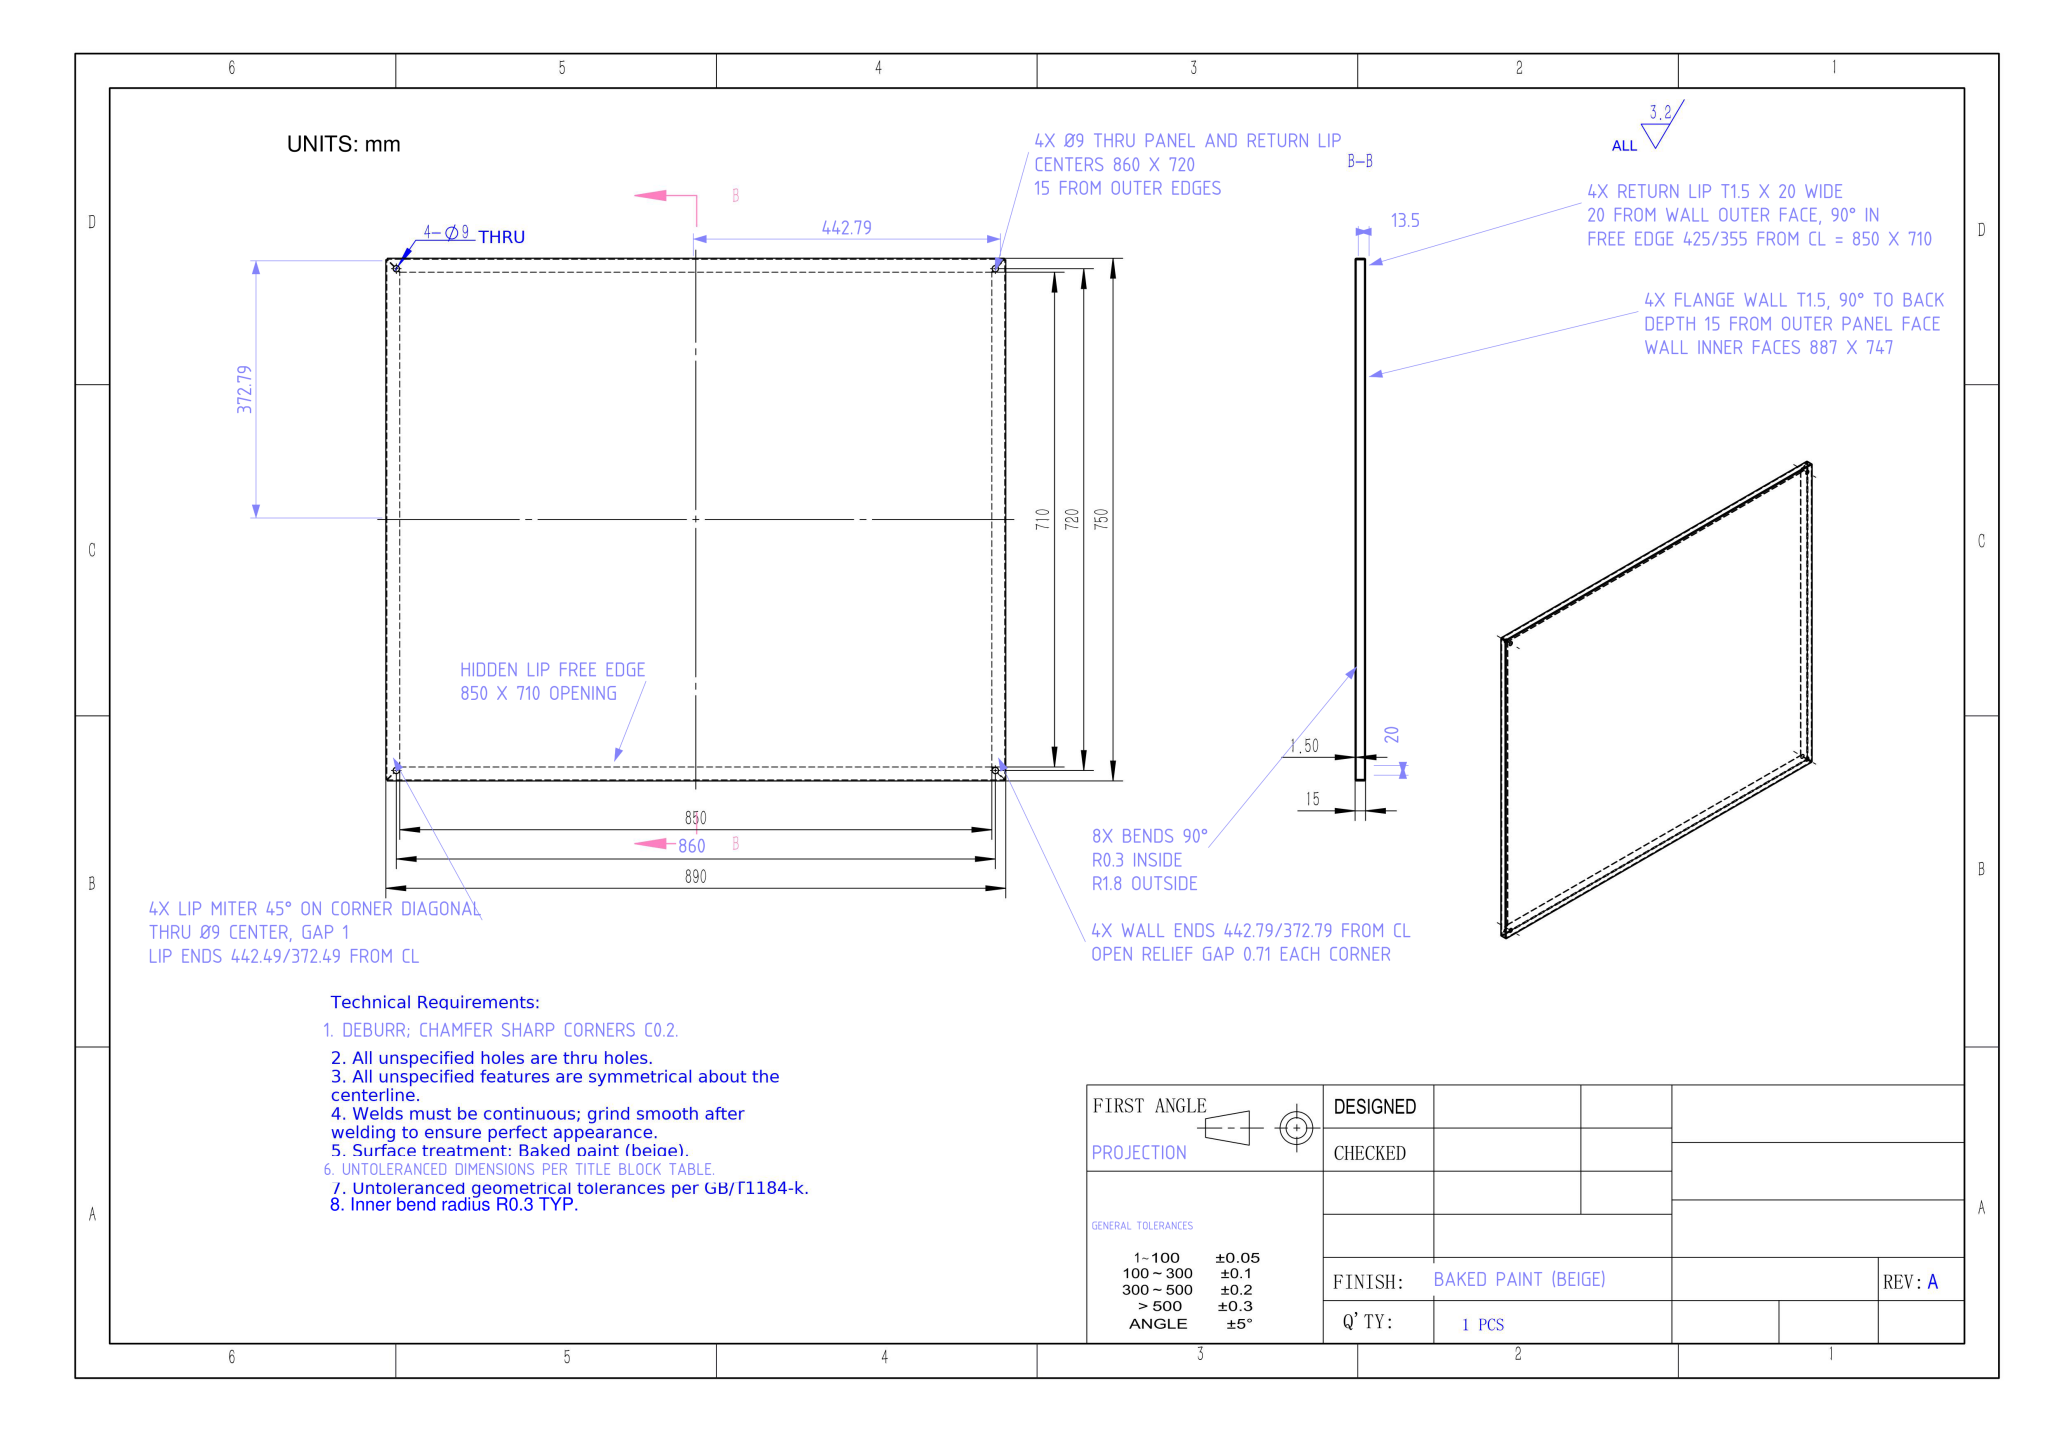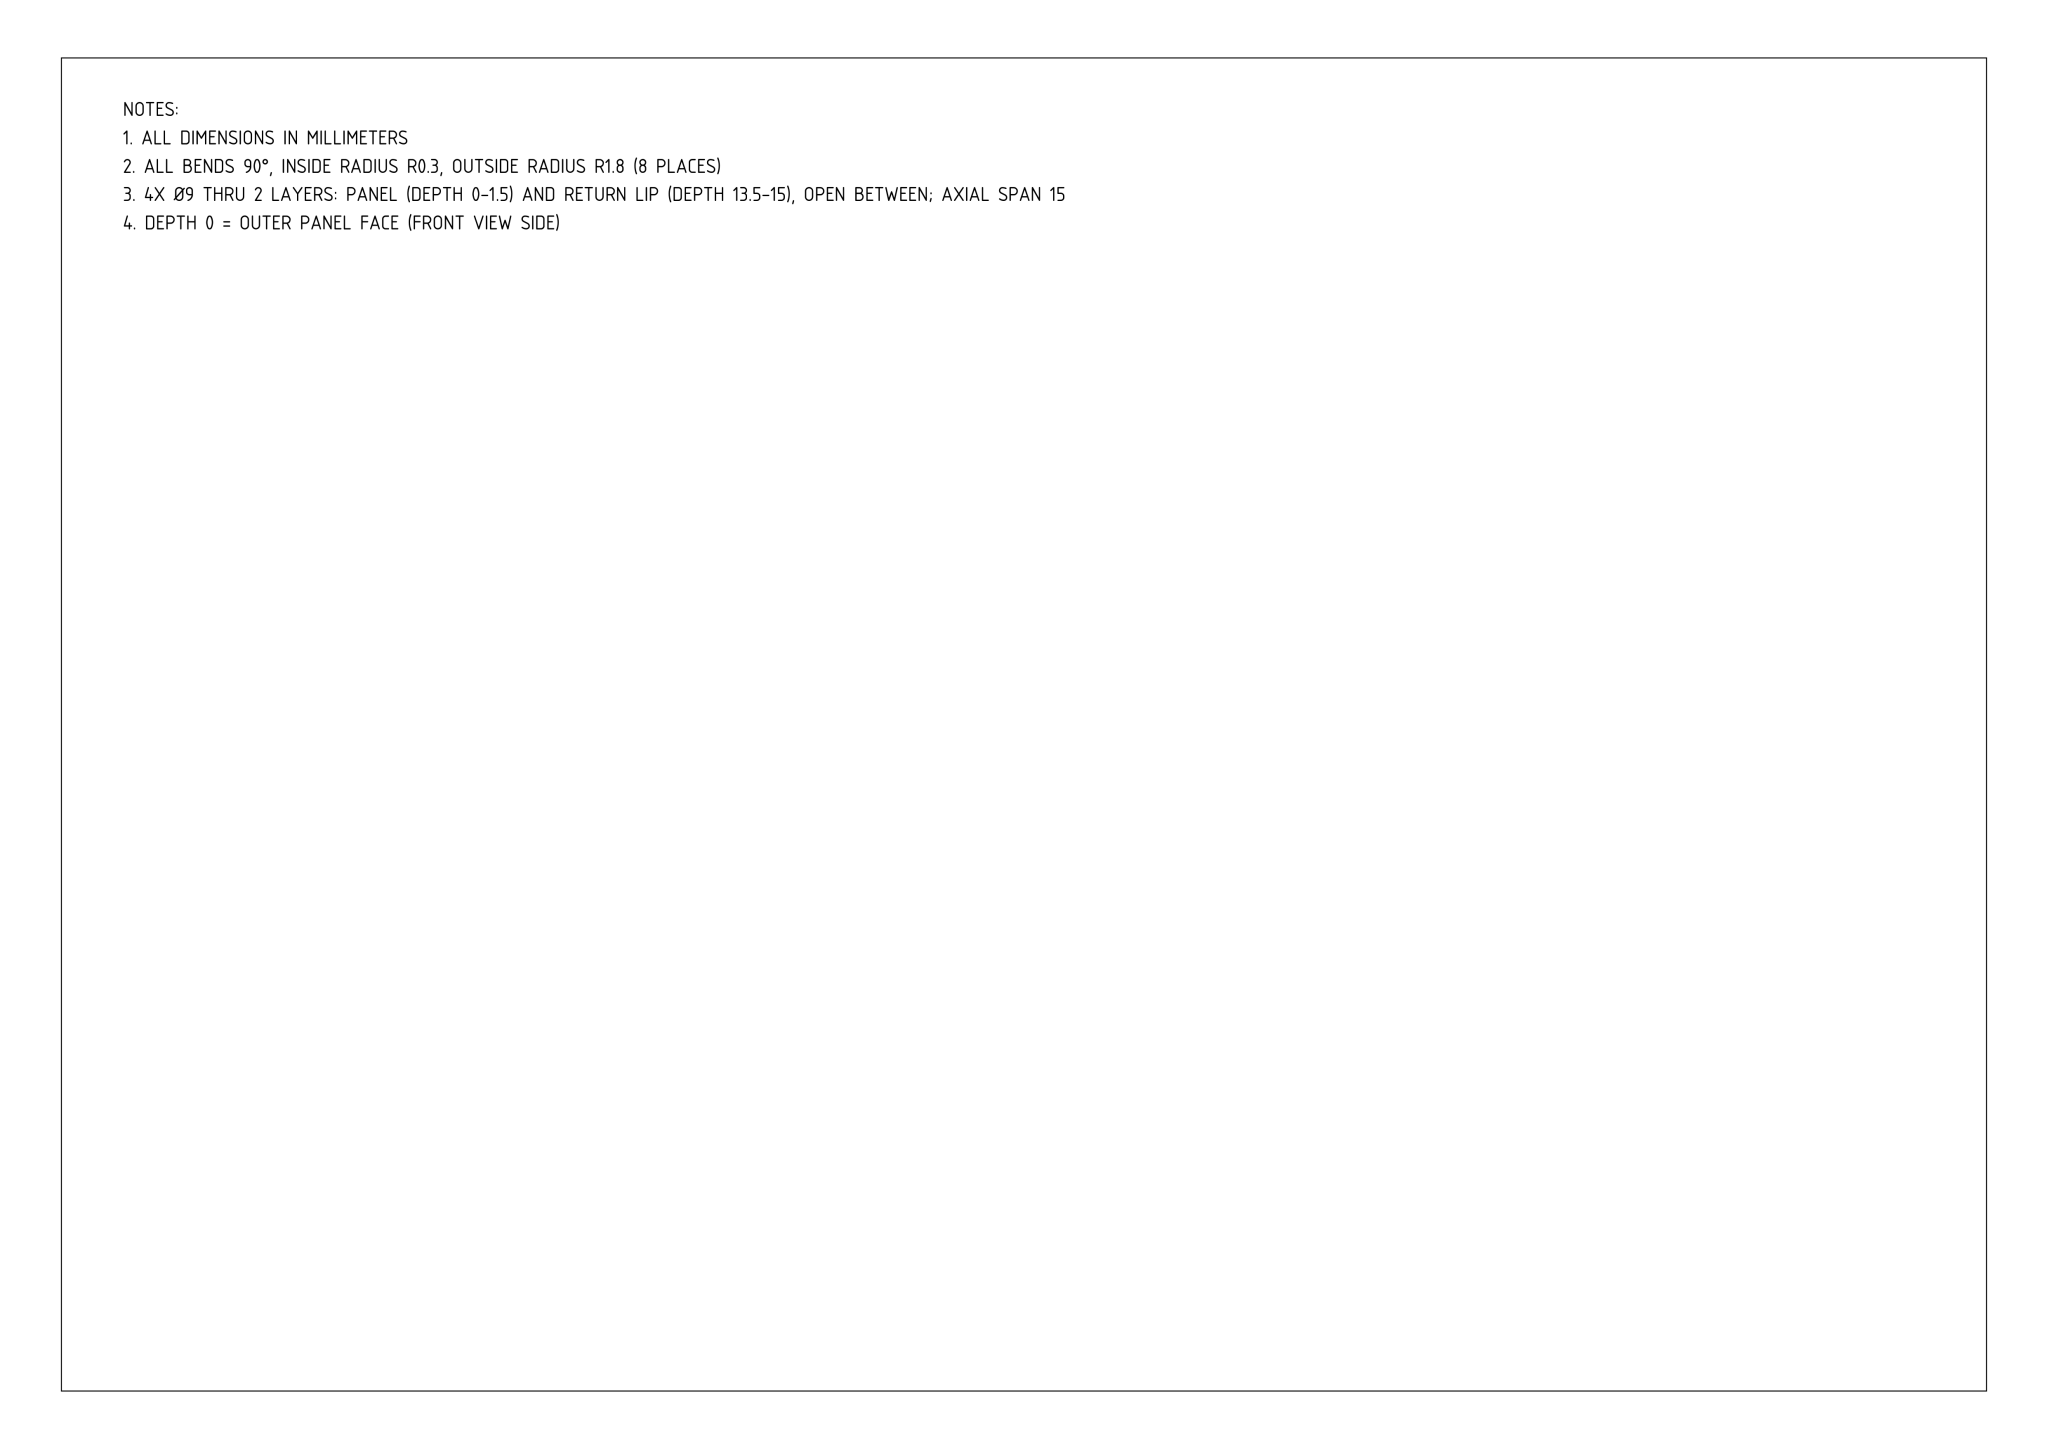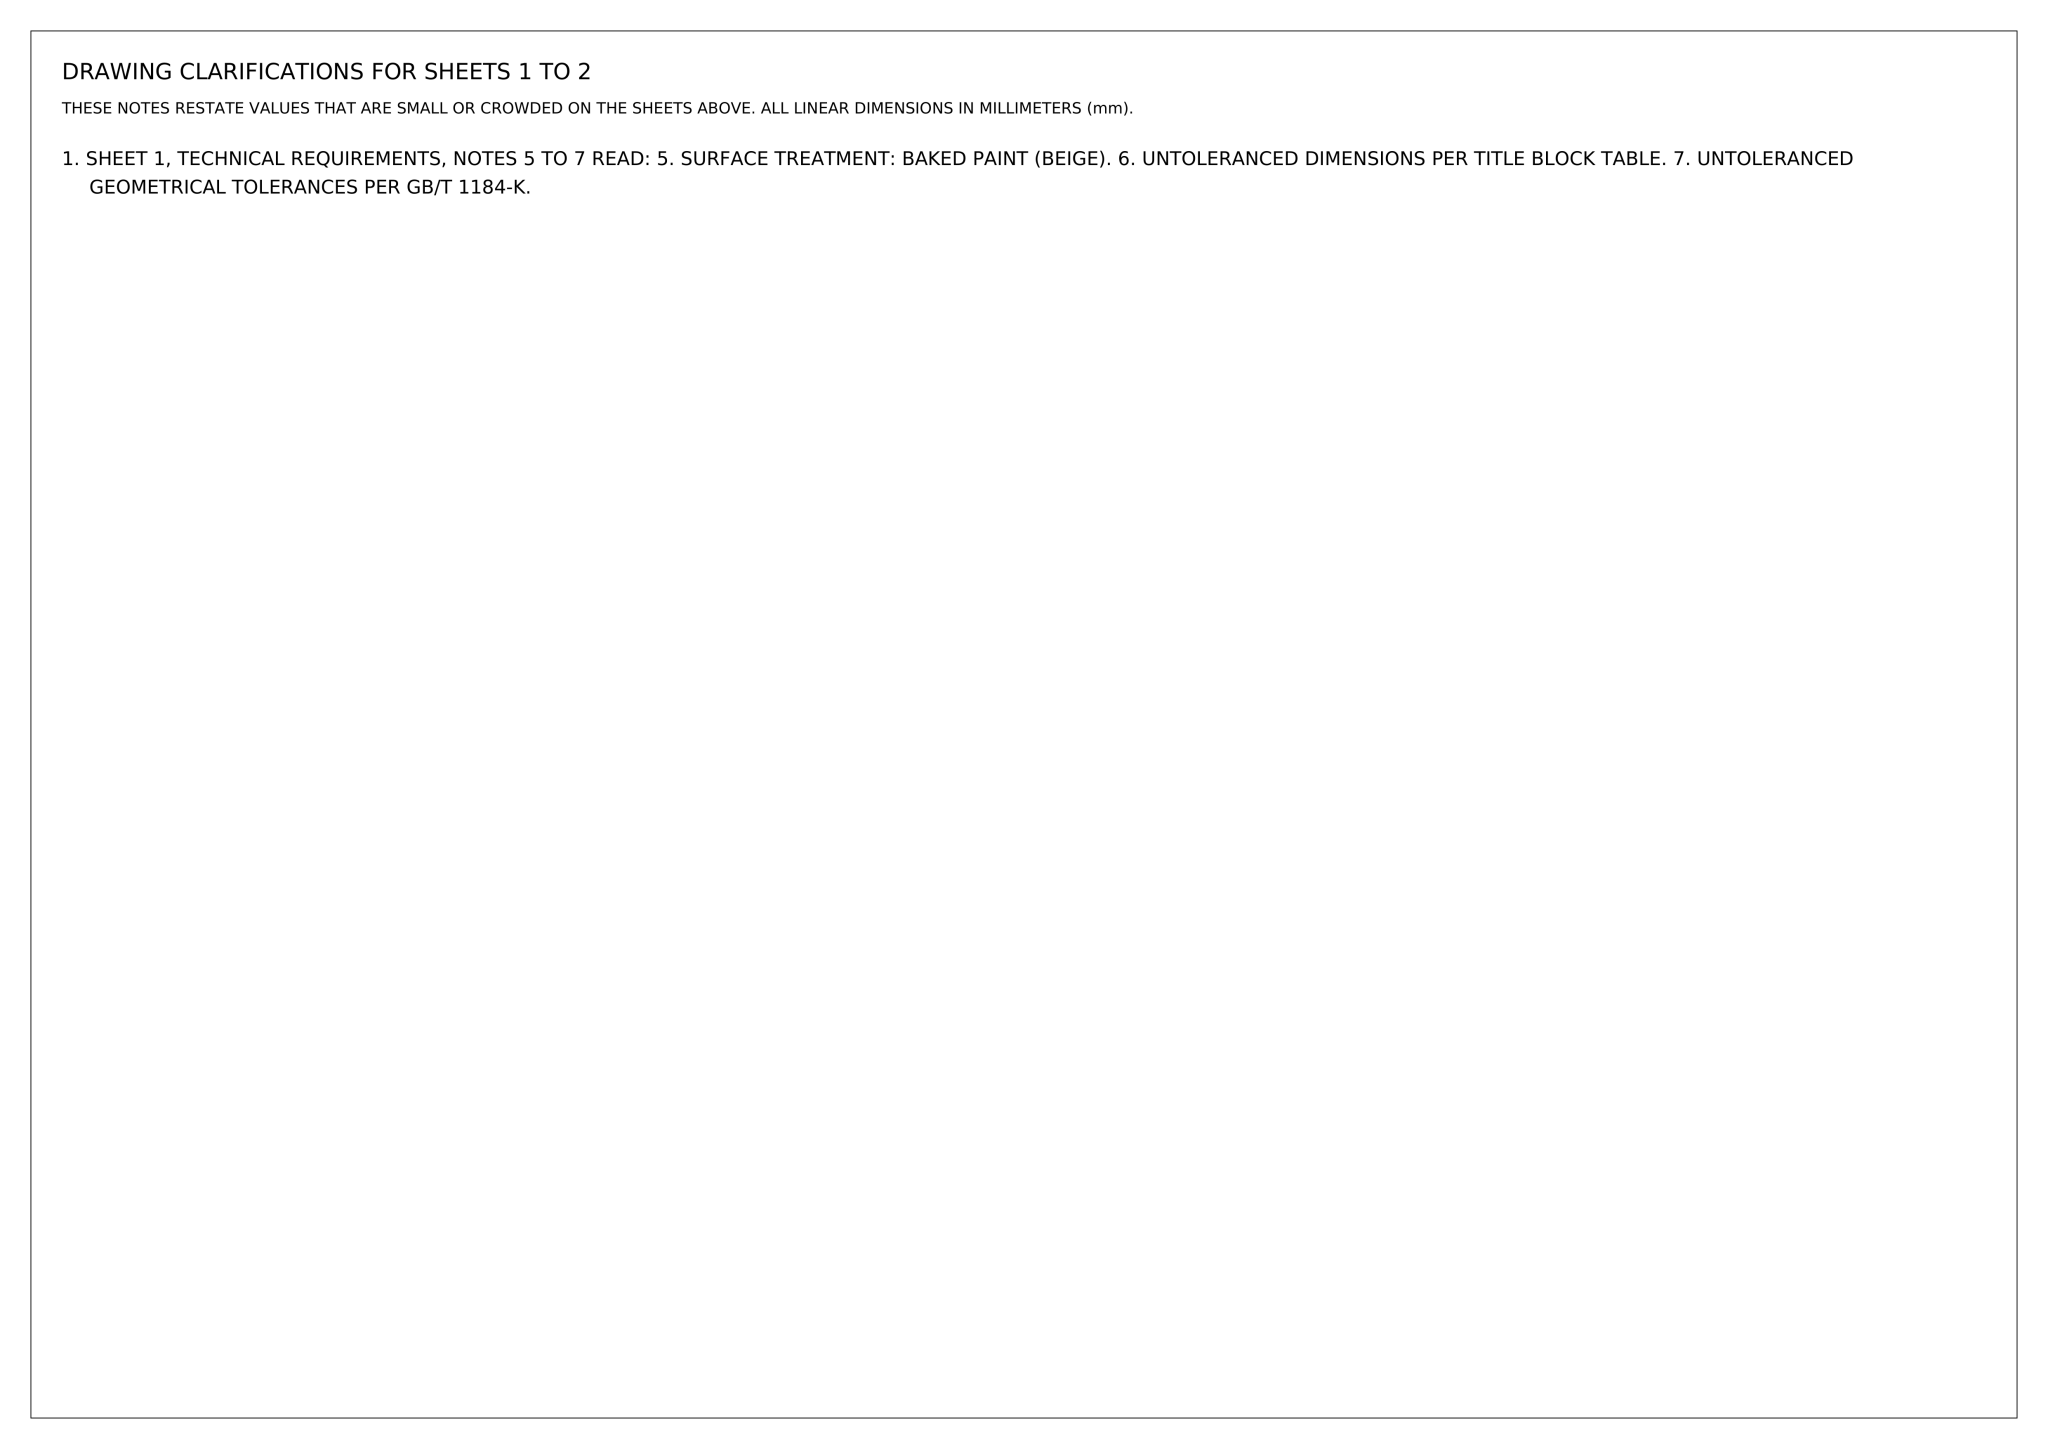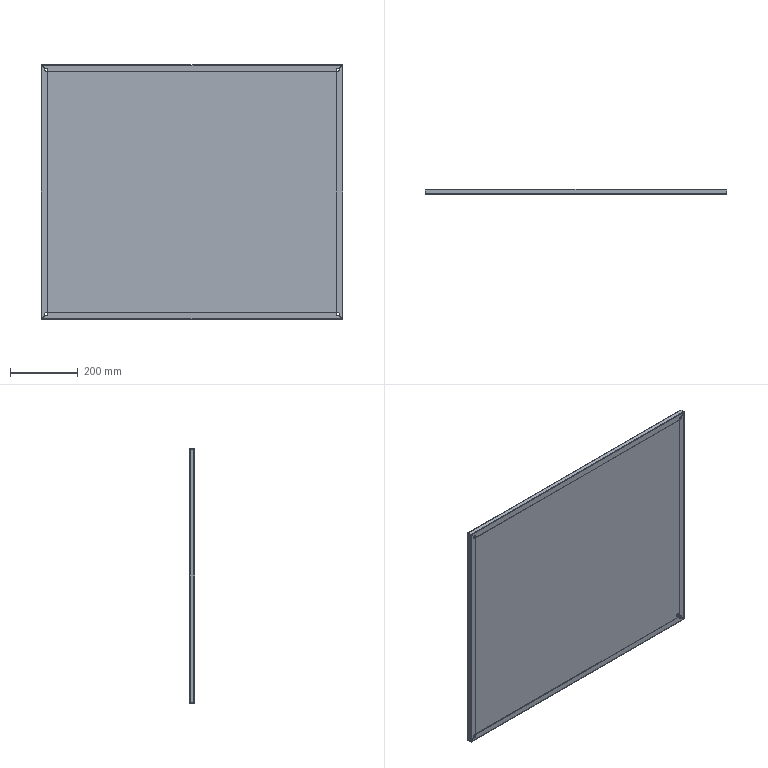Part | NX | mm | 1 solid | 98 faces | box 890 x 15 x 750 mm | volume 1150642 mm3 | plane 46 | cylinder 36 | spline 16 | commonest cylinder face diameters 9 x20 3.6 x8 0.6 x8